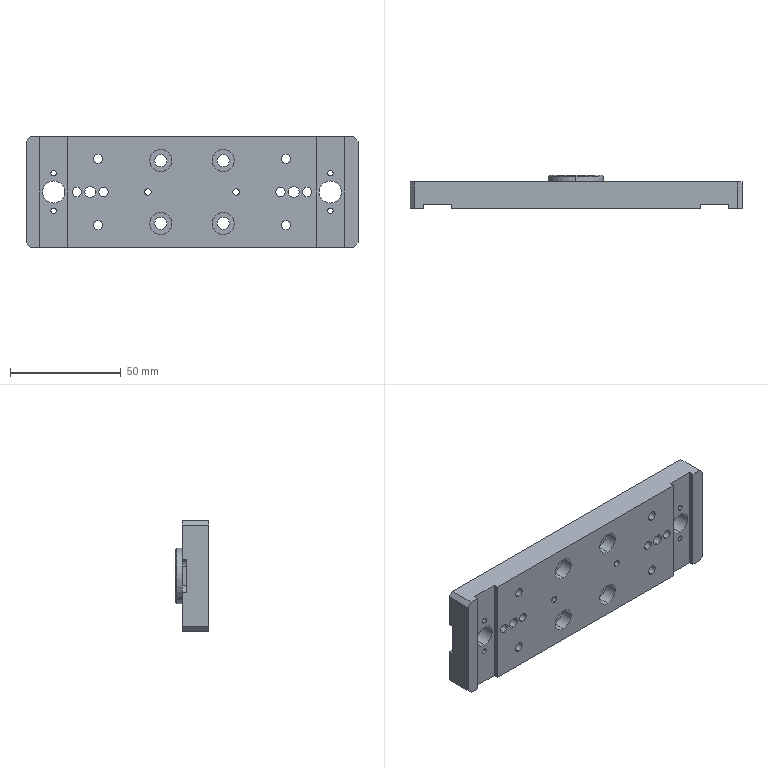Component | SolidWorks | F-SZP17248-10-03-1 | 1 solid | 95 faces | box 150 x 15 x 50 mm | volume 80560 mm3 | cylinder 58 | plane 35 | cone 2 | commonest cylinder face diameters 4.2 x16 10 x12 5.5 x8 2.5 x8 5 x4 3 x4 6 x4 25 x2
build123d program:
from build123d import *

# Parameters (mm, degrees)
SKETCH1_W                                          = 150
SKETCH1_H                                          = 50
BOSS_EXTRUDE1_DEPTH                                = 6
SKETCH2_R                                          = 12.5
BOSS_EXTRUDE2_DEPTH                                = 3
CHAMFER1_SIZE                                      = 0.5
HOLE_SIZE_ACCORDING_TO_TYPE_OF_HEXAGON_D           = 5.5
HOLE_SIZE_ACCORDING_TO_TYPE_OF_HEXAGON_CBORE_D     = 10
HOLE_SIZE_ACCORDING_TO_TYPE_OF_HEXAGON_CBORE_DEPTH = 5.7
SKETCH5_R                                          = 1.5
CUT_EXTRUDE1_DEPTH                                 = 81.467
CHAMFER2_SIZE                                      = 2
SKETCH6_R                                          = 5
CUT_EXTRUDE2_DEPTH                                 = 80.962
M3_TAPPED_HOLE1_D                                  = 2.5
M5_TAPPED_HOLE1_D                                  = 4.2
SKETCH12_W                                         = 45
SKETCH12_H                                         = 15
CUT_EXTRUDE4_DEPTH                                 = 2
FILLET1_R                                          = 3
M5_TAPPED_HOLE2_D                                  = 4.2
SKETCH15_W                                         = 12.5
SKETCH15_H                                         = 50
SKETCH15_R                                         = 1.25
SKETCH15_R_2                                       = 5
CUT_EXTRUDE5_DEPTH                                 = 2
SKETCH16_R                                         = 2.5
CUT_EXTRUDE6_DEPTH                                 = 24


with BuildPart() as part:
    # Sketch1 → Boss-Extrude1 (new, symmetric)
    with BuildSketch(Plane(origin=(0, 0, 0), x_dir=(1, 0, 0), z_dir=(0, 1, 0))):
        Rectangle(SKETCH1_W, SKETCH1_H)
    extrude(amount=BOSS_EXTRUDE1_DEPTH, both=True)

    # Sketch2 → Boss-Extrude2 (add)
    with BuildSketch(Plane(origin=(0, 6, 0), x_dir=(1, 0, 0), z_dir=(0, 1, 0))):
        with Locations(Location((0, 0, 0), (0, 0, 90))):
            Circle(SKETCH2_R)
    extrude(amount=BOSS_EXTRUDE2_DEPTH)

    # Chamfer1
    chamfer1_edges = [part.edges().sort_by_distance(p)[0] for p in [
        (0, 9, 12.5),
    ]]
    chamfer(chamfer1_edges, length=CHAMFER1_SIZE)

    # Hole Size_According to_ Type of Hexagon (through all)
    with Locations(Plane(origin=(0, -6, 0), x_dir=(-1, 0, 0), z_dir=(0, -1, 0))):
        with Locations((-14.142, -14.142), (-14.142, 14.142), (14.142, 14.142), (14.142, -14.142)):
            CounterBoreHole(HOLE_SIZE_ACCORDING_TO_TYPE_OF_HEXAGON_D / 2, HOLE_SIZE_ACCORDING_TO_TYPE_OF_HEXAGON_CBORE_D / 2, HOLE_SIZE_ACCORDING_TO_TYPE_OF_HEXAGON_CBORE_DEPTH)

    # Sketch5 → Cut-Extrude1 (cut, through all)
    with BuildSketch(Plane.XZ.offset(6)):
        with Locations(Location((20, 0, 0), (0, 0, 270))):
            Circle(SKETCH5_R)
        with Locations(Location((-20, 0, 0), (0, 0, 270))):
            Circle(SKETCH5_R)
    extrude(amount=-CUT_EXTRUDE1_DEPTH, mode=Mode.SUBTRACT)

    # Chamfer2
    chamfer2_edges = [part.edges().sort_by_distance(p)[0] for p in [
        (75, 0, 25),
        (-75, 0, 25),
        (-75, 0, -25),
        (75, 0, -25),
    ]]
    chamfer(chamfer2_edges, length=CHAMFER2_SIZE)

    # Sketch6 → Cut-Extrude2 (cut, through all)
    with BuildSketch(Plane(origin=(0, 6, 0), x_dir=(1, 0, 0), z_dir=(0, 1, 0))):
        with Locations(Location((-62.5, 0, 0), (0, 0, 270))):
            Circle(SKETCH6_R)
        with Locations(Location((62.5, 0, 0), (0, 0, 270))):
            Circle(SKETCH6_R)
    extrude(amount=-CUT_EXTRUDE2_DEPTH, mode=Mode.SUBTRACT)

    # M3 Tapped Hole1 (through all)
    with Locations(Plane(origin=(0, 6, 0), x_dir=(1, 0, 0), z_dir=(0, 1, 0))):
        with Locations((-62.5, 8.5), (-62.5, -8.5), (62.5, 8.5), (62.5, -8.5)):
            Hole(M3_TAPPED_HOLE1_D / 2)

    # M5 Tapped Hole1 (through all)
    with Locations(Plane(origin=(0, -6, 0), x_dir=(-1, 0, 0), z_dir=(0, -1, 0))):
        with Locations((42.5, -15), (42.5, 15)):
            m5_tapped_hole1 = Hole(M5_TAPPED_HOLE1_D / 2)

    # Mirror1: M5 Tapped Hole1 across plane
    add(m5_tapped_hole1.mirror(Plane(origin=(0, 0, 0), x_dir=(0, 0, 1), z_dir=(1, 0, 0))), mode=Mode.SUBTRACT)

    # Sketch12 → Cut-Extrude4 (cut)
    with BuildSketch(Plane(origin=(0, 6, 0), x_dir=(1, 0, 0), z_dir=(0, 1, 0))):
        with Locations((52.5, 0)):
            Rectangle(SKETCH12_W, SKETCH12_H)
        with Locations((-52.5, 0)):
            Rectangle(SKETCH12_W, SKETCH12_H)
    extrude(amount=-CUT_EXTRUDE4_DEPTH, mode=Mode.SUBTRACT)

    # Fillet1
    fillet1_edges = [part.edges().sort_by_distance(p)[0] for p in [
        (30, 5, -7.5),
        (30, 5, 7.5),
        (-30, 5, 7.5),
        (-30, 5, -7.5),
    ]]
    fillet(fillet1_edges, radius=FILLET1_R)

    # M5 Tapped Hole2 (through all)
    with Locations(Plane(origin=(0, 4, 0), x_dir=(1, 0, 0), z_dir=(0, 1, 0))):
        with Locations((40, 0), (52, 0)):
            m5_tapped_hole2 = Hole(M5_TAPPED_HOLE2_D / 2)

    # Mirror2: M5 Tapped Hole2 across plane
    add(m5_tapped_hole2.mirror(Plane(origin=(0, 0, 0), x_dir=(0, 0, 1), z_dir=(1, 0, 0))), mode=Mode.SUBTRACT)

    # Sketch15 → Cut-Extrude5 (cut)
    # profile 1 of 2: a face of its own
    with BuildSketch(Plane.XZ.offset(6)):
        with Locations((-62.5, 0)):
            Rectangle(SKETCH15_W, SKETCH15_H)
        with Locations(Location((-62.5, -8.5, 0), (0, 0, 53.13))):
            Circle(SKETCH15_R, mode=Mode.SUBTRACT)
        with Locations(Location((-62.5, 0, 0), (0, 0, 90))):
            Circle(SKETCH15_R_2, mode=Mode.SUBTRACT)
        with Locations(Location((-62.5, 8.5, 0), (0, 0, 233.13))):
            Circle(SKETCH15_R, mode=Mode.SUBTRACT)
    # profile 2 of 2: a face of its own
    with BuildSketch(Plane.XZ.offset(6)):
        with Locations((62.5, 0)):
            Rectangle(SKETCH15_W, SKETCH15_H)
        with Locations(Location((62.5, -8.5, 0), (0, 0, 53.13))):
            Circle(SKETCH15_R, mode=Mode.SUBTRACT)
        with Locations(Location((62.5, 0, 0), (0, 0, 90))):
            Circle(SKETCH15_R_2, mode=Mode.SUBTRACT)
        with Locations(Location((62.5, 8.5, 0), (0, 0, 233.13))):
            Circle(SKETCH15_R, mode=Mode.SUBTRACT)
    extrude(amount=-CUT_EXTRUDE5_DEPTH, mode=Mode.SUBTRACT)

    # Sketch16 → Cut-Extrude6 (cut)
    with BuildSketch(Plane(origin=(0, 6, 0), x_dir=(1, 0, 0), z_dir=(0, 1, 0))):
        with Locations(Location((-46, 0, 0), (0, 0, 270))):
            Circle(SKETCH16_R)
        with Locations(Location((46, 0, 0), (0, 0, 270))):
            Circle(SKETCH16_R)
    extrude(amount=-CUT_EXTRUDE6_DEPTH, mode=Mode.SUBTRACT)


solid = part.part

# Placed as in the assembly
solid = solid.moved(Location((-45.188, -24.343, 123.72), (0, 0, 0)))